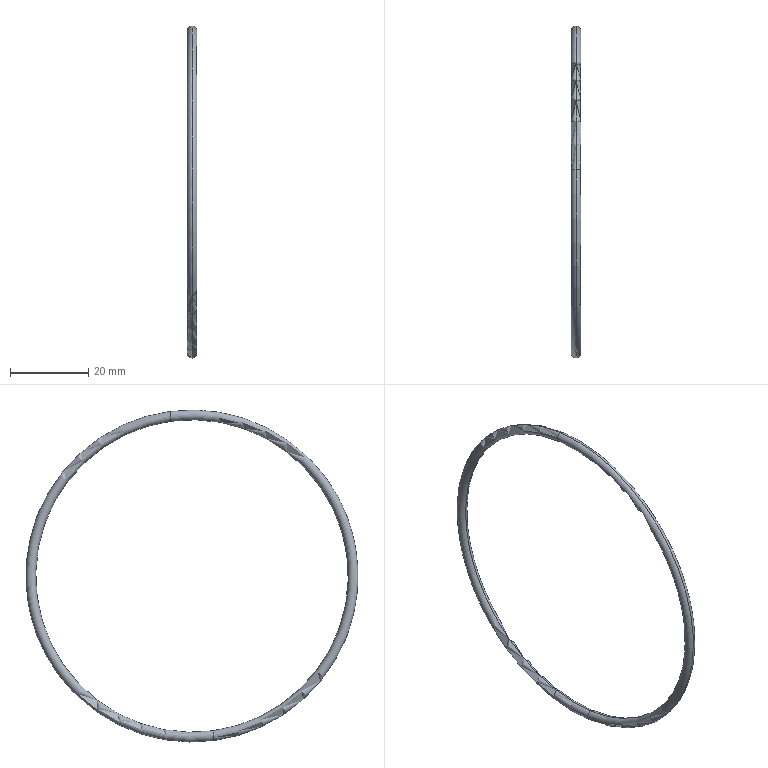Component | SolidWorks | 11O-ring-1 | 1 solid | 4 faces | box 2.5 x 85 x 85 mm | volume 1272 mm3 | torus 4
build123d program:
from build123d import *

# Parameters (mm, degrees)
SWEEP1_PROFILE_R = 1.25


with BuildPart() as part:
    # Sweep1: sweep along a path in Sketch8
    with BuildLine(Plane.XY) as sweep1_path:
        CenterArc((0, 0), 41.25, 0, 360)
    # Sweep1 profile (on start of the path) → Sweep1 (sweep)
    with BuildSketch(Plane(origin=(41.25, 0, 0), x_dir=(0, 0, 1), z_dir=(0, 1, 0))):
        Circle(SWEEP1_PROFILE_R)
    sweep(path=sweep1_path.line)


solid = part.part

# Placed as in the assembly
solid = solid.moved(Location((224.41, -90.191, 512), (0, 90, 0)))
STEP:
#1=CARTESIAN_POINT('',(8.835,-3.329,21.816));
#2=VERTEX_POINT('',#1);
#3=CARTESIAN_POINT('',(8.835,-3.342,21.718));
#4=VERTEX_POINT('',#3);
#5=CARTESIAN_POINT('',(8.835,-3.335,21.767));
#6=DIRECTION('',(0.,0.9912,-0.1327));
#7=DIRECTION('',(0.,0.1327,0.9912));
#8=AXIS2_PLACEMENT_3D('',#5,#6,#7);
#9=CIRCLE('',#8,0.04921);
#10=EDGE_CURVE('',#2,#4,#9,.T.);
#11=ORIENTED_EDGE('',*,*,#10,.F.);
#12=CARTESIAN_POINT('',(8.835,-3.773,18.499));
#13=VERTEX_POINT('',#12);
#14=CARTESIAN_POINT('',(8.835,-3.551,20.157));
#15=DIRECTION('',(1.,0.,0.));
#16=DIRECTION('',(0.,0.,-1.));
#17=AXIS2_PLACEMENT_3D('',#14,#15,#16);
#18=CIRCLE('',#17,1.673);
#19=EDGE_CURVE('',#2,#13,#18,.T.);
#20=ORIENTED_EDGE('',*,*,#19,.T.);
#21=CARTESIAN_POINT('',(8.835,-3.76,18.597));
#22=VERTEX_POINT('',#21);
#23=CARTESIAN_POINT('',(8.835,-3.766,18.548));
#24=DIRECTION('',(0.,-0.9912,0.1327));
#25=DIRECTION('',(0.,-0.1327,-0.9912));
#26=AXIS2_PLACEMENT_3D('',#23,#24,#25);
#27=CIRCLE('',#26,0.04921);
#28=EDGE_CURVE('',#13,#22,#27,.T.);
#29=ORIENTED_EDGE('',*,*,#28,.T.);
#30=CARTESIAN_POINT('',(8.835,-3.551,20.157));
#31=DIRECTION('',(1.,0.,0.));
#32=DIRECTION('',(0.,0.,-1.));
#33=AXIS2_PLACEMENT_3D('',#30,#31,#32);
#34=CIRCLE('',#33,1.575);
#35=EDGE_CURVE('',#4,#22,#34,.T.);
#36=ORIENTED_EDGE('',*,*,#35,.F.);
#37=EDGE_LOOP('',(#11,#20,#29,#36));
#38=FACE_OUTER_BOUND('',#37,.T.);
#39=CARTESIAN_POINT('',(8.835,-3.551,20.157));
#40=DIRECTION('',(1.,0.,0.));
#41=DIRECTION('',(0.,-0.1327,-0.9912));
#42=AXIS2_PLACEMENT_3D('',#39,#40,#41);
#43=TOROIDAL_SURFACE('',#42,1.624,0.04921);
#44=ADVANCED_FACE('',(#38),#43,.T.);
#45=ORIENTED_EDGE('',*,*,#28,.F.);
#46=CARTESIAN_POINT('',(8.835,-3.551,20.157));
#47=DIRECTION('',(1.,0.,0.));
#48=DIRECTION('',(0.,0.,-1.));
#49=AXIS2_PLACEMENT_3D('',#46,#47,#48);
#50=CIRCLE('',#49,1.673);
#51=EDGE_CURVE('',#13,#2,#50,.T.);
#52=ORIENTED_EDGE('',*,*,#51,.T.);
#53=ORIENTED_EDGE('',*,*,#10,.T.);
#54=CARTESIAN_POINT('',(8.835,-3.551,20.157));
#55=DIRECTION('',(1.,0.,0.));
#56=DIRECTION('',(0.,0.,-1.));
#57=AXIS2_PLACEMENT_3D('',#54,#55,#56);
#58=CIRCLE('',#57,1.575);
#59=EDGE_CURVE('',#22,#4,#58,.T.);
#60=ORIENTED_EDGE('',*,*,#59,.F.);
#61=EDGE_LOOP('',(#45,#52,#53,#60));
#62=FACE_OUTER_BOUND('',#61,.T.);
#63=CARTESIAN_POINT('',(8.835,-3.551,20.157));
#64=DIRECTION('',(1.,0.,0.));
#65=DIRECTION('',(0.,-0.1327,-0.9912));
#66=AXIS2_PLACEMENT_3D('',#63,#64,#65);
#67=TOROIDAL_SURFACE('',#66,1.624,0.04921);
#68=ADVANCED_FACE('',(#62),#67,.T.);
#69=ORIENTED_EDGE('',*,*,#51,.F.);
#70=CARTESIAN_POINT('',(8.835,-3.766,18.548));
#71=DIRECTION('',(0.,-0.9912,0.1327));
#72=DIRECTION('',(0.,-0.1327,-0.9912));
#73=AXIS2_PLACEMENT_3D('',#70,#71,#72);
#74=CIRCLE('',#73,0.04921);
#75=EDGE_CURVE('',#22,#13,#74,.T.);
#76=ORIENTED_EDGE('',*,*,#75,.F.);
#77=ORIENTED_EDGE('',*,*,#59,.T.);
#78=CARTESIAN_POINT('',(8.835,-3.335,21.767));
#79=DIRECTION('',(0.,0.9912,-0.1327));
#80=DIRECTION('',(0.,0.1327,0.9912));
#81=AXIS2_PLACEMENT_3D('',#78,#79,#80);
#82=CIRCLE('',#81,0.04921);
#83=EDGE_CURVE('',#4,#2,#82,.T.);
#84=ORIENTED_EDGE('',*,*,#83,.T.);
#85=EDGE_LOOP('',(#69,#76,#77,#84));
#86=FACE_OUTER_BOUND('',#85,.T.);
#87=CARTESIAN_POINT('',(8.835,-3.551,20.157));
#88=DIRECTION('',(1.,0.,0.));
#89=DIRECTION('',(0.,-0.1327,-0.9912));
#90=AXIS2_PLACEMENT_3D('',#87,#88,#89);
#91=TOROIDAL_SURFACE('',#90,1.624,0.04921);
#92=ADVANCED_FACE('',(#86),#91,.T.);
#93=ORIENTED_EDGE('',*,*,#19,.F.);
#94=ORIENTED_EDGE('',*,*,#83,.F.);
#95=ORIENTED_EDGE('',*,*,#35,.T.);
#96=ORIENTED_EDGE('',*,*,#75,.T.);
#97=EDGE_LOOP('',(#93,#94,#95,#96));
#98=FACE_OUTER_BOUND('',#97,.T.);
#99=CARTESIAN_POINT('',(8.835,-3.551,20.157));
#100=DIRECTION('',(1.,0.,0.));
#101=DIRECTION('',(0.,-0.1327,-0.9912));
#102=AXIS2_PLACEMENT_3D('',#99,#100,#101);
#103=TOROIDAL_SURFACE('',#102,1.624,0.04921);
#104=ADVANCED_FACE('',(#98),#103,.T.);
#105=CLOSED_SHELL('',(#44,#68,#92,#104));
#106=MANIFOLD_SOLID_BREP('',#105);
#107=CARTESIAN_POINT('',(0.,0.,0.));
#108=DIRECTION('',(0.,0.,1.));
#109=DIRECTION('',(1.,0.,0.));
#110=AXIS2_PLACEMENT_3D('',#107,#108,#109);
#111=(LENGTH_UNIT()NAMED_UNIT(*)SI_UNIT($,.METRE.));
#112=LENGTH_MEASURE_WITH_UNIT(LENGTH_MEASURE(0.0254),#111);
#113=DIMENSIONAL_EXPONENTS(1.,0.,0.,0.,0.,0.,0.);
#114=(CONVERSION_BASED_UNIT('',#112)LENGTH_UNIT()NAMED_UNIT(#113));
#115=UNCERTAINTY_MEASURE_WITH_UNIT(LENGTH_MEASURE(0.00001),#114,'','');
#116=(NAMED_UNIT(*)PLANE_ANGLE_UNIT()SI_UNIT($,.RADIAN.));
#117=(NAMED_UNIT(*)SI_UNIT($,.STERADIAN.)SOLID_ANGLE_UNIT());
#118=(GEOMETRIC_REPRESENTATION_CONTEXT(3)GLOBAL_UNCERTAINTY_ASSIGNED_CONTEXT((#115))GLOBAL_UNIT_ASSIGNED_CONTEXT((#114,#116,#117))REPRESENTATION_CONTEXT('',''));
#119=ADVANCED_BREP_SHAPE_REPRESENTATION('',(#106,#110),#118);
#120=COLOUR_RGB('',0.7922,0.8196,0.9333);
#121=FILL_AREA_STYLE_COLOUR('',#120);
#122=FILL_AREA_STYLE('',(#121));
#123=SURFACE_STYLE_FILL_AREA(#122);
#124=SURFACE_SIDE_STYLE('',(#123));
#125=SURFACE_STYLE_USAGE(.BOTH.,#124);
#126=PRESENTATION_STYLE_ASSIGNMENT((#125));
#127=STYLED_ITEM('',(#126),#106);
#128=(LENGTH_UNIT()NAMED_UNIT(*)SI_UNIT($,.METRE.));
#129=LENGTH_MEASURE_WITH_UNIT(LENGTH_MEASURE(0.0254),#128);
#130=DIMENSIONAL_EXPONENTS(1.,0.,0.,0.,0.,0.,0.);
#131=(CONVERSION_BASED_UNIT('',#129)LENGTH_UNIT()NAMED_UNIT(#130));
#132=UNCERTAINTY_MEASURE_WITH_UNIT(LENGTH_MEASURE(0.00001),#131,'','');
#133=(NAMED_UNIT(*)PLANE_ANGLE_UNIT()SI_UNIT($,.RADIAN.));
#134=(NAMED_UNIT(*)SI_UNIT($,.STERADIAN.)SOLID_ANGLE_UNIT());
#135=(GEOMETRIC_REPRESENTATION_CONTEXT(3)GLOBAL_UNCERTAINTY_ASSIGNED_CONTEXT((#132))GLOBAL_UNIT_ASSIGNED_CONTEXT((#131,#133,#134))REPRESENTATION_CONTEXT('',''));
#136=MECHANICAL_DESIGN_GEOMETRIC_PRESENTATION_REPRESENTATION('',(#127),#135);
#137=PRESENTATION_LAYER_ASSIGNMENT('','',(#127));